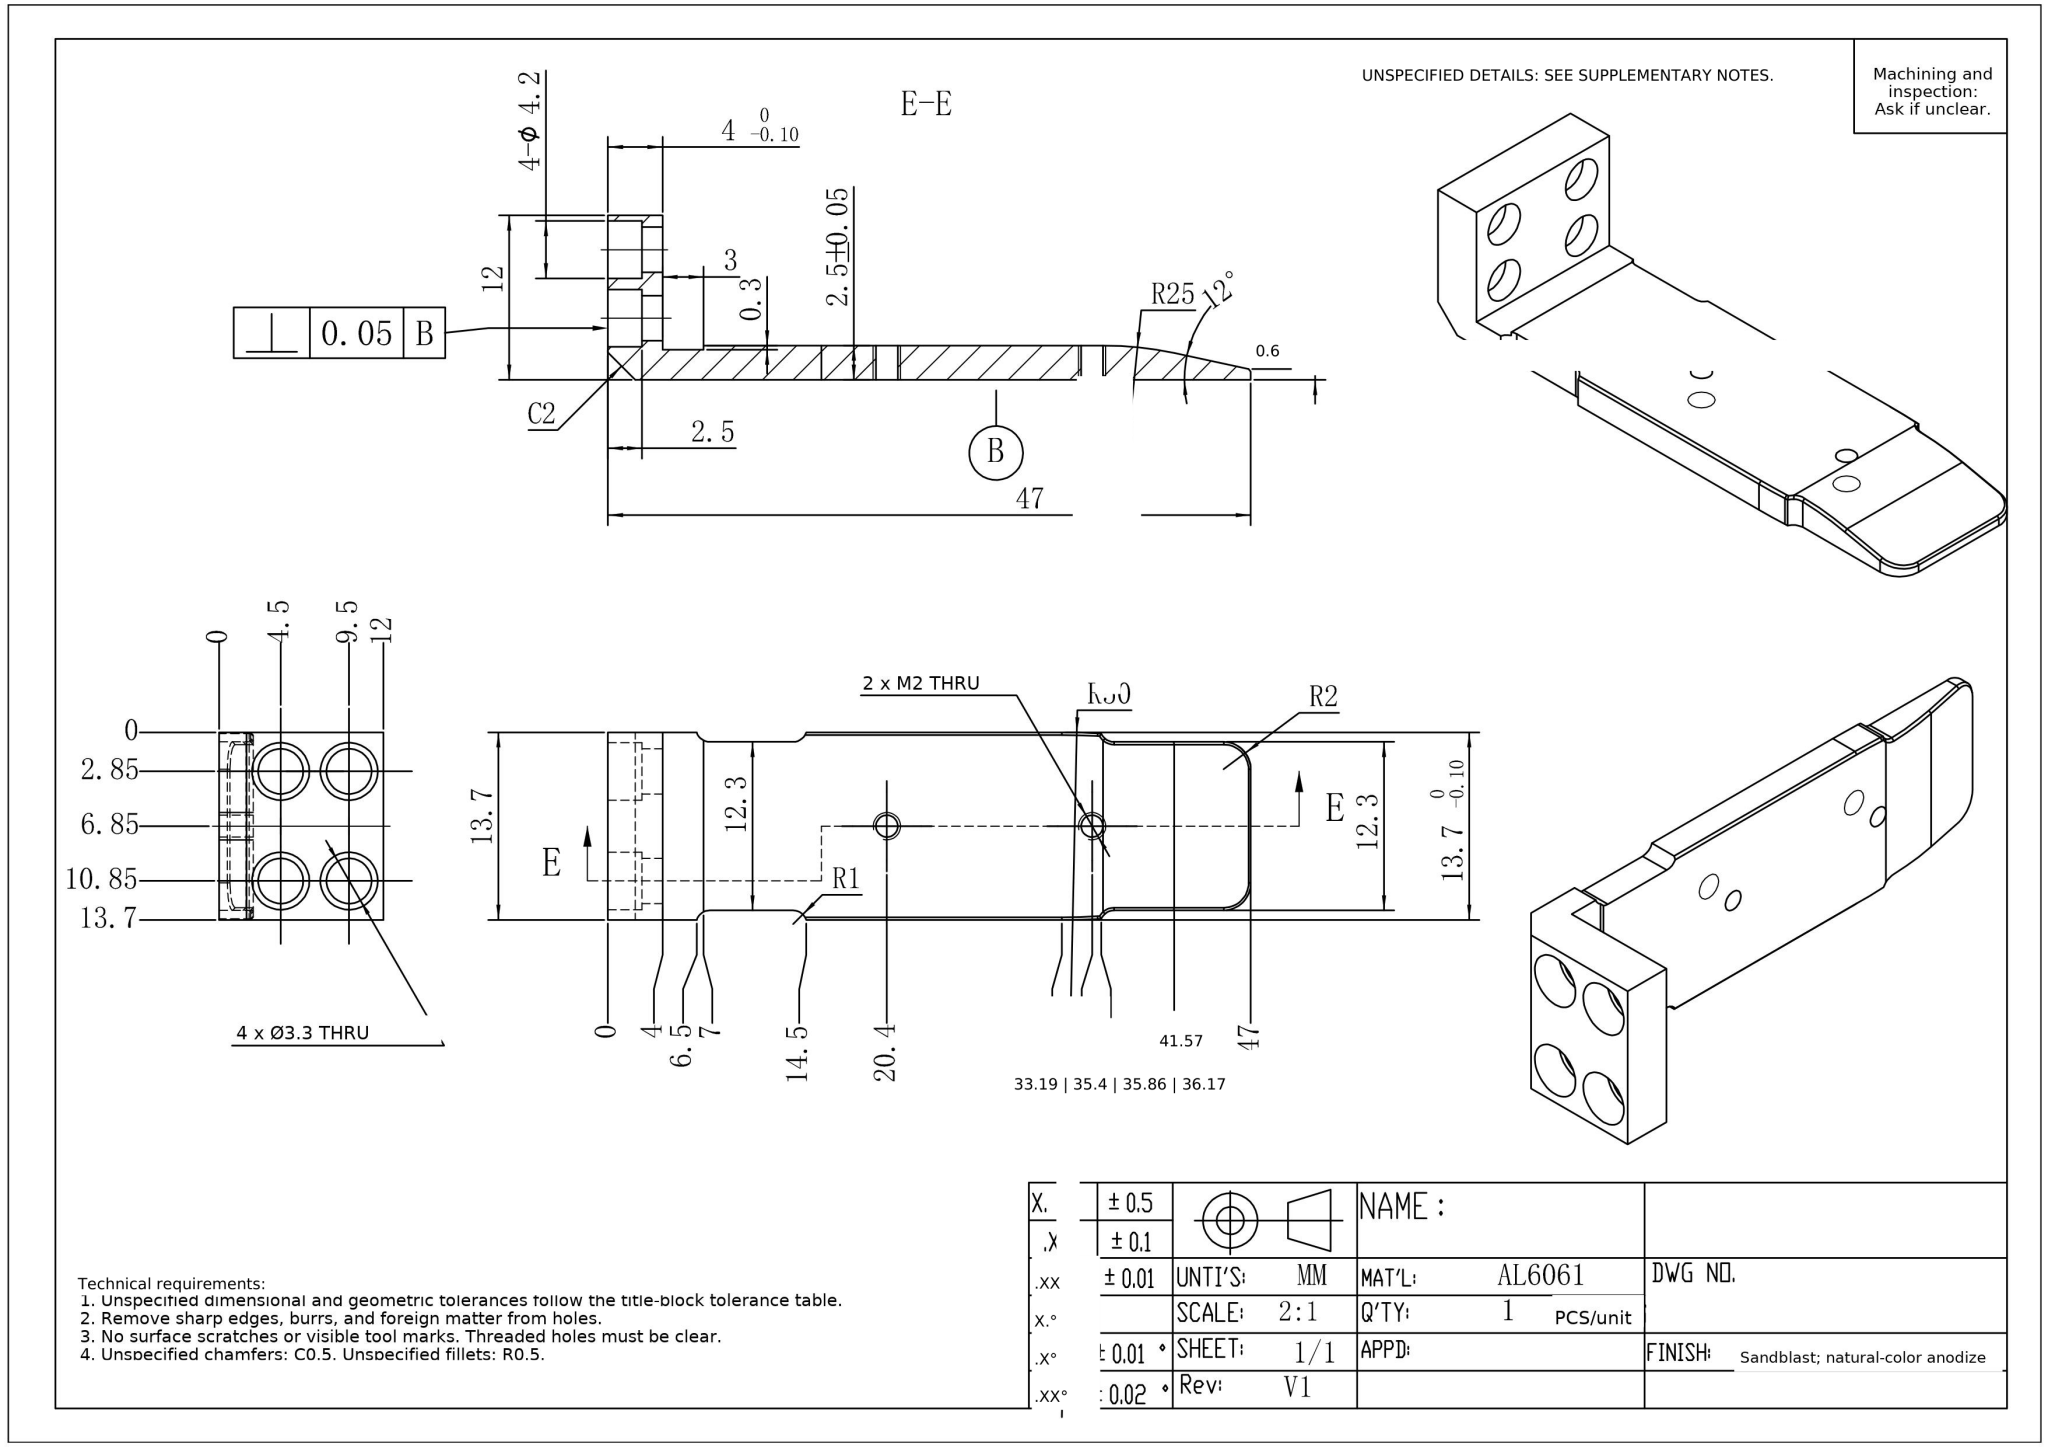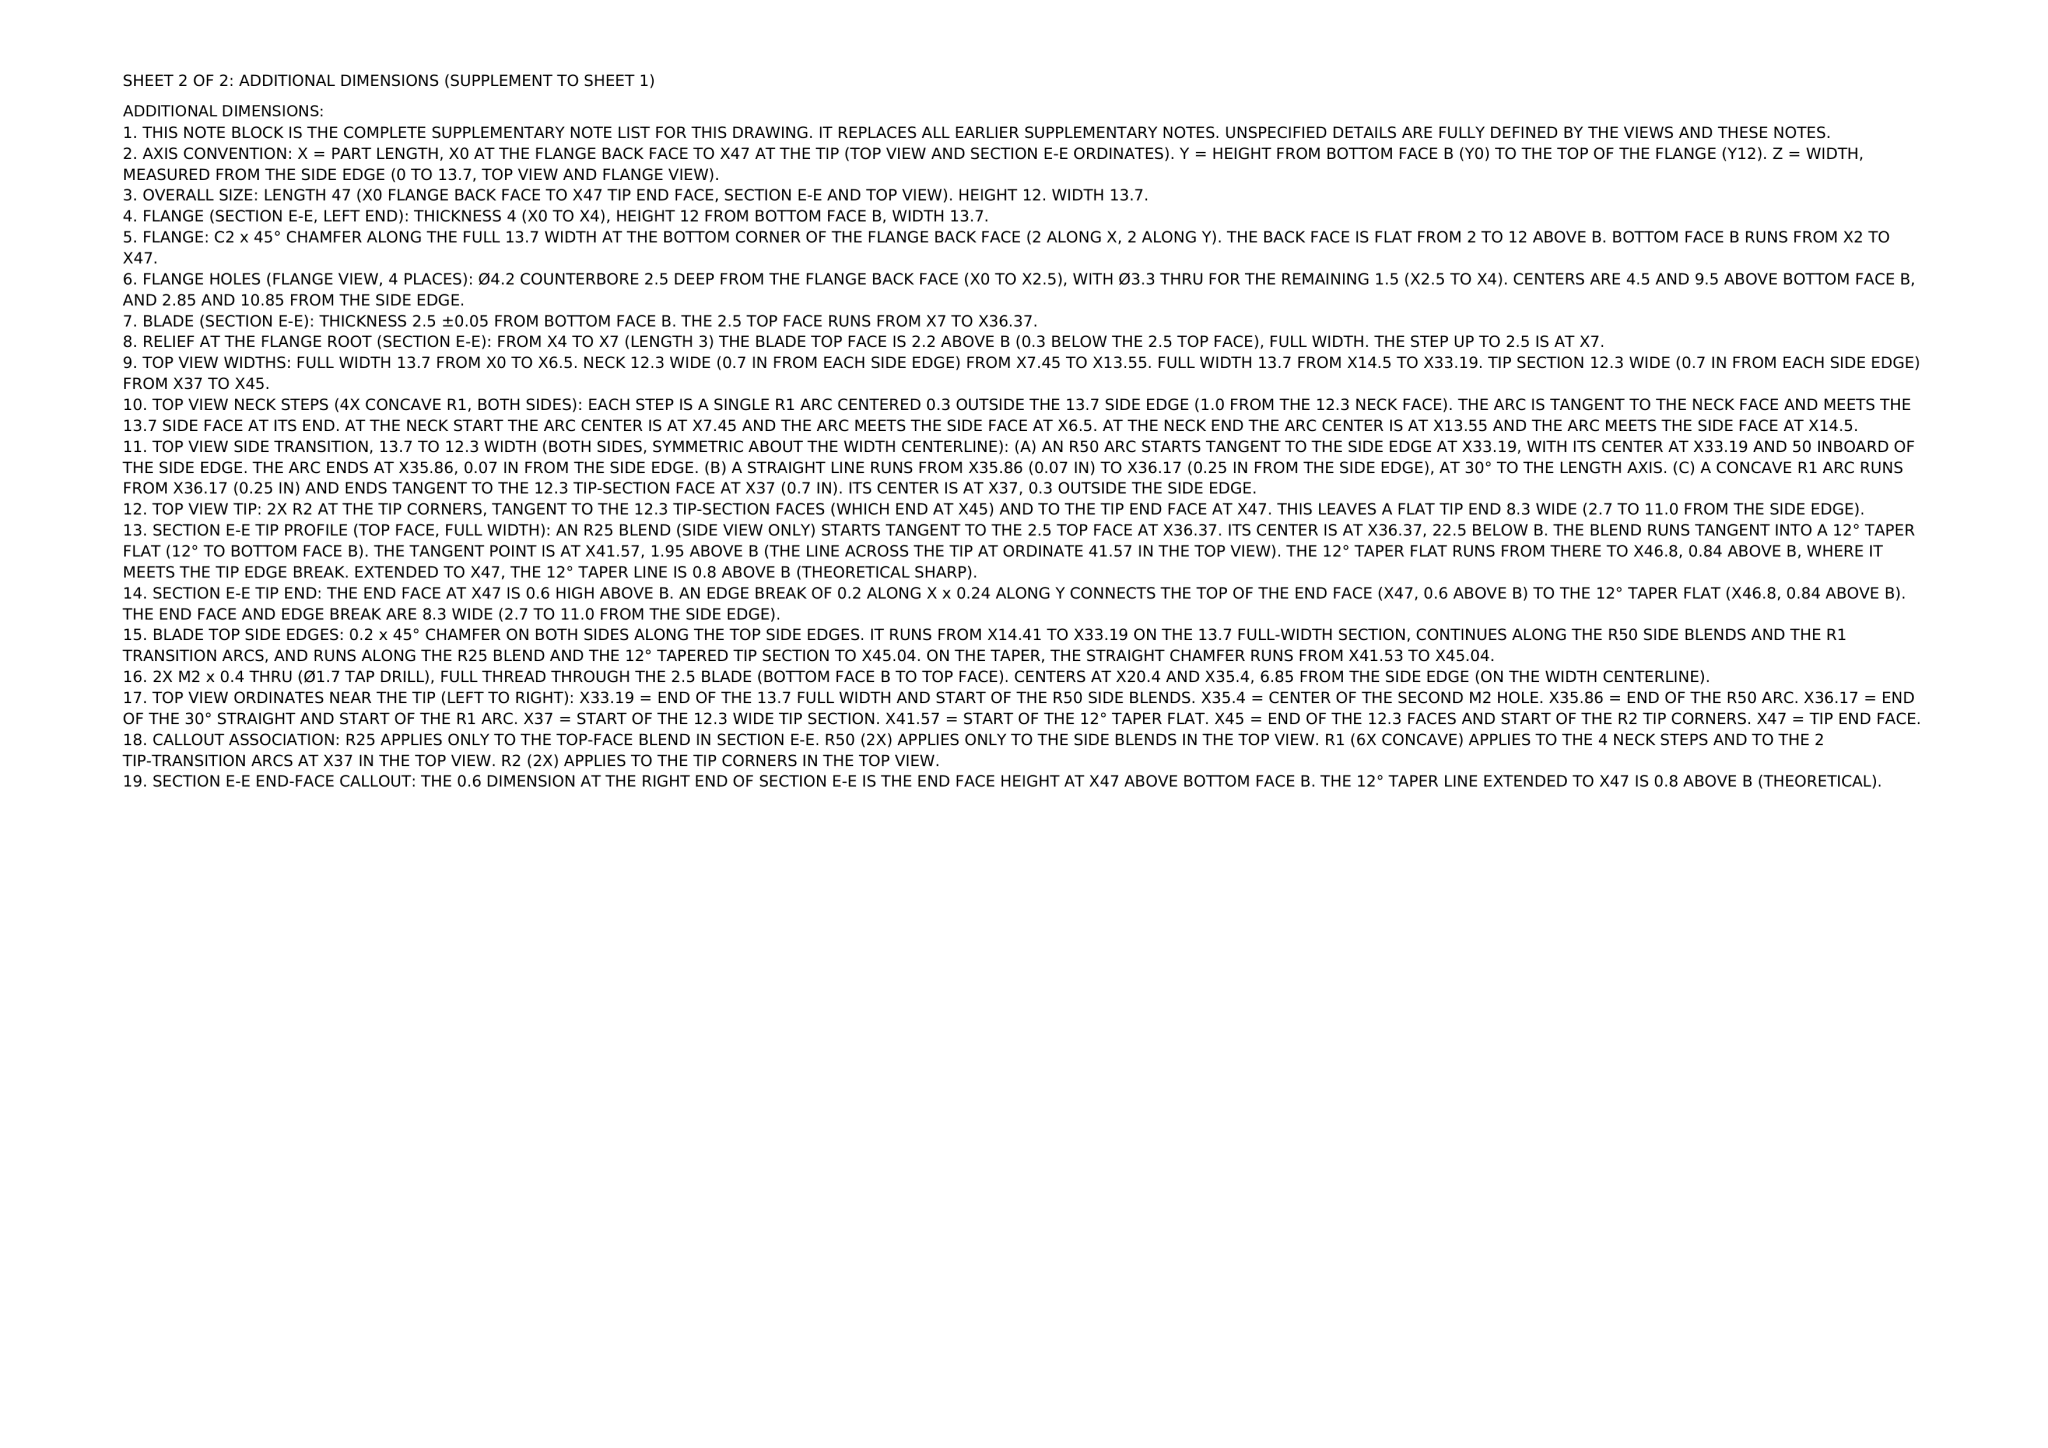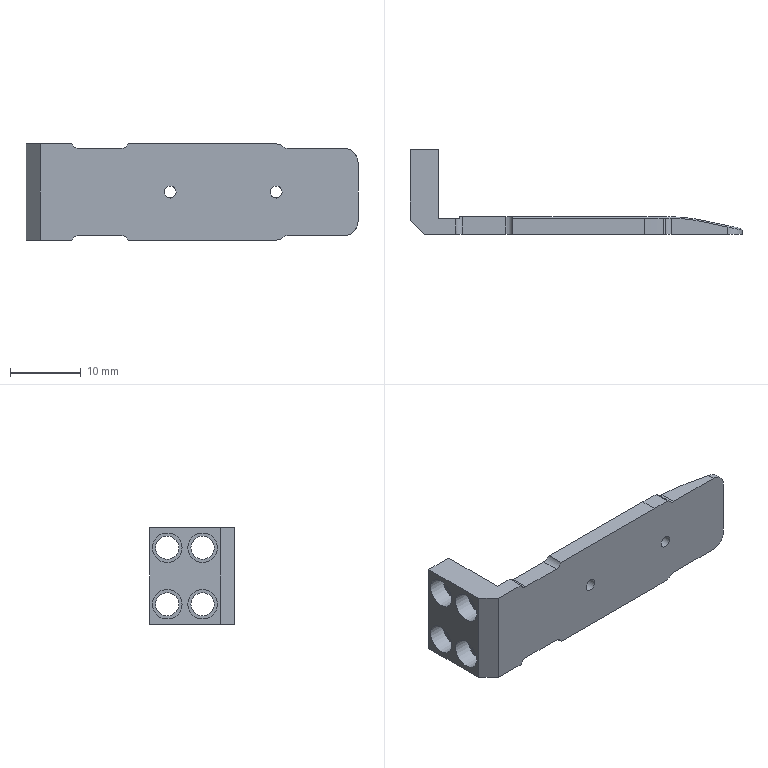Part | NX | mm | 1 solid | 62 faces | box 47 x 12 x 13.7 mm | volume 1736 mm3 | plane 29 | cylinder 21 | cone 6 | spline 6 | commonest cylinder face diameters 2 x6 3.3 x4 4.2 x4 1.7 x2 100 x2 4 x2 50 x1